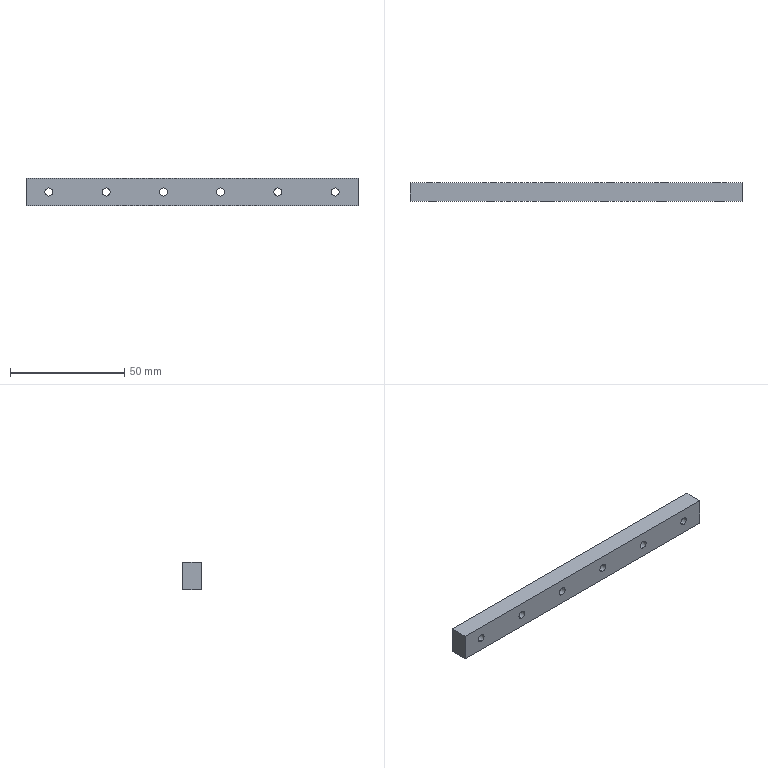Component | SolidWorks | MGN12H1R145Z0C-1_MGN12H145-1 | 1 solid | 36 faces | box 145 x 8 x 12 mm | volume 12955 mm3 | cylinder 24 | plane 12 | commonest cylinder face diameters 3.5 x12 6 x12 | material Plain Carbon Steel
build123d program:
from build123d import *

# Parameters (mm, degrees)
SKETCH1_W                                       = 12
SKETCH1_H                                       = 8
EXTRUDE1_DEPTH                                  = 145
M3_HEX_SOCKET_HEAD_CAP_SCREW_CBORE1_D           = 3.5
M3_HEX_SOCKET_HEAD_CAP_SCREW_CBORE1_CBORE_D     = 6
M3_HEX_SOCKET_HEAD_CAP_SCREW_CBORE1_CBORE_DEPTH = 4.5
LPATTERN1_COUNT                                 = 6
LPATTERN1_PITCH                                 = 25


with BuildPart() as part:
    # Sketch1 → Extrude1 (new body)
    with BuildSketch(Plane(origin=(0, 0, 0), x_dir=(0, 0, -1), z_dir=(1, 0, 0))):
        with Locations((0, 4)):
            Rectangle(SKETCH1_W, SKETCH1_H)
    extrude(amount=EXTRUDE1_DEPTH)

    # M3 Hex Socket Head Cap Screw CBORE1 (through all)
    with Locations(Plane(origin=(135, 8, 0), x_dir=(0, 0, 1), z_dir=(0, 1, 0))):
        with Locations((0, 0)):
            m3_hex_socket_head_cap_screw_cbore1 = CounterBoreHole(M3_HEX_SOCKET_HEAD_CAP_SCREW_CBORE1_D / 2, M3_HEX_SOCKET_HEAD_CAP_SCREW_CBORE1_CBORE_D / 2, M3_HEX_SOCKET_HEAD_CAP_SCREW_CBORE1_CBORE_DEPTH)

    # LPattern1: M3 Hex Socket Head Cap Screw CBORE1 ×6
    with Locations(*[(-i * LPATTERN1_PITCH, 0, 0) for i in range(1, LPATTERN1_COUNT)]):
        add(m3_hex_socket_head_cap_screw_cbore1, mode=Mode.SUBTRACT)


solid = part.part

# Placed as in the assembly
solid = solid.moved(Location((-3.73, 8.768, 38.329), (0, 0, 0)))
STEP:
#1=COLOUR_RGB('',0.7922,0.8196,0.9333);
#2=FILL_AREA_STYLE_COLOUR('',#1);
#3=FILL_AREA_STYLE('',(#2));
#4=SURFACE_STYLE_FILL_AREA(#3);
#5=SURFACE_SIDE_STYLE('',(#4));
#6=SURFACE_STYLE_USAGE(.BOTH.,#5);
#7=PRESENTATION_STYLE_ASSIGNMENT((#6));
#8=CARTESIAN_POINT('',(0.2469,0.3452,1.44));
#9=VERTEX_POINT('',#8);
#10=CARTESIAN_POINT('',(0.2469,0.3452,1.578));
#11=VERTEX_POINT('',#10);
#12=CARTESIAN_POINT('',(0.2469,0.3452,1.509));
#13=DIRECTION('',(0.,1.,0.));
#14=DIRECTION('',(0.,0.,1.));
#15=AXIS2_PLACEMENT_3D('',#12,#13,#14);
#16=CIRCLE('',#15,0.0689);
#17=EDGE_CURVE('',#9,#11,#16,.T.);
#18=ORIENTED_EDGE('',*,*,#17,.F.);
#19=CARTESIAN_POINT('',(0.2469,0.483,1.44));
#20=VERTEX_POINT('',#19);
#21=CARTESIAN_POINT('',(0.2469,0.6602,1.44));
#22=DIRECTION('',(0.,1.,0.));
#23=VECTOR('',#22,39.37);
#24=LINE('',#21,#23);
#25=EDGE_CURVE('',#9,#20,#24,.T.);
#26=ORIENTED_EDGE('',*,*,#25,.T.);
#27=CARTESIAN_POINT('',(0.2469,0.483,1.578));
#28=VERTEX_POINT('',#27);
#29=CARTESIAN_POINT('',(0.2469,0.483,1.509));
#30=DIRECTION('',(0.,1.,0.));
#31=DIRECTION('',(0.,0.,1.));
#32=AXIS2_PLACEMENT_3D('',#29,#30,#31);
#33=CIRCLE('',#32,0.0689);
#34=EDGE_CURVE('',#20,#28,#33,.T.);
#35=ORIENTED_EDGE('',*,*,#34,.T.);
#36=CARTESIAN_POINT('',(0.2469,0.6602,1.578));
#37=DIRECTION('',(0.,1.,0.));
#38=VECTOR('',#37,39.37);
#39=LINE('',#36,#38);
#40=EDGE_CURVE('',#11,#28,#39,.T.);
#41=ORIENTED_EDGE('',*,*,#40,.F.);
#42=EDGE_LOOP('',(#18,#26,#35,#41));
#43=FACE_OUTER_BOUND('',#42,.T.);
#44=CARTESIAN_POINT('',(0.2469,0.6602,1.509));
#45=DIRECTION('',(0.,1.,0.));
#46=DIRECTION('',(0.,0.,1.));
#47=AXIS2_PLACEMENT_3D('',#44,#45,#46);
#48=CYLINDRICAL_SURFACE('',#47,0.0689);
#49=ADVANCED_FACE('',(#43),#48,.F.);
#50=CARTESIAN_POINT('',(0.2469,0.483,1.391));
#51=VERTEX_POINT('',#50);
#52=CARTESIAN_POINT('',(0.2469,0.483,1.627));
#53=VERTEX_POINT('',#52);
#54=CARTESIAN_POINT('',(0.2469,0.483,1.509));
#55=DIRECTION('',(0.,1.,0.));
#56=DIRECTION('',(0.,0.,1.));
#57=AXIS2_PLACEMENT_3D('',#54,#55,#56);
#58=CIRCLE('',#57,0.1181);
#59=EDGE_CURVE('',#51,#53,#58,.T.);
#60=ORIENTED_EDGE('',*,*,#59,.F.);
#61=CARTESIAN_POINT('',(0.2469,0.6602,1.391));
#62=VERTEX_POINT('',#61);
#63=CARTESIAN_POINT('',(0.2469,0.6602,1.391));
#64=DIRECTION('',(0.,1.,0.));
#65=VECTOR('',#64,39.37);
#66=LINE('',#63,#65);
#67=EDGE_CURVE('',#51,#62,#66,.T.);
#68=ORIENTED_EDGE('',*,*,#67,.T.);
#69=CARTESIAN_POINT('',(0.2469,0.6602,1.627));
#70=VERTEX_POINT('',#69);
#71=CARTESIAN_POINT('',(0.2469,0.6602,1.509));
#72=DIRECTION('',(0.,1.,0.));
#73=DIRECTION('',(0.,0.,1.));
#74=AXIS2_PLACEMENT_3D('',#71,#72,#73);
#75=CIRCLE('',#74,0.1181);
#76=EDGE_CURVE('',#62,#70,#75,.T.);
#77=ORIENTED_EDGE('',*,*,#76,.T.);
#78=CARTESIAN_POINT('',(0.2469,0.6602,1.627));
#79=DIRECTION('',(0.,1.,0.));
#80=VECTOR('',#79,39.37);
#81=LINE('',#78,#80);
#82=EDGE_CURVE('',#53,#70,#81,.T.);
#83=ORIENTED_EDGE('',*,*,#82,.F.);
#84=EDGE_LOOP('',(#60,#68,#77,#83));
#85=FACE_OUTER_BOUND('',#84,.T.);
#86=CARTESIAN_POINT('',(0.2469,0.6602,1.509));
#87=DIRECTION('',(0.,1.,0.));
#88=DIRECTION('',(0.,0.,1.));
#89=AXIS2_PLACEMENT_3D('',#86,#87,#88);
#90=CYLINDRICAL_SURFACE('',#89,0.1181);
#91=ADVANCED_FACE('',(#85),#90,.F.);
#92=CARTESIAN_POINT('',(1.231,0.3452,1.44));
#93=VERTEX_POINT('',#92);
#94=CARTESIAN_POINT('',(1.231,0.3452,1.578));
#95=VERTEX_POINT('',#94);
#96=CARTESIAN_POINT('',(1.231,0.3452,1.509));
#97=DIRECTION('',(0.,1.,0.));
#98=DIRECTION('',(0.,0.,1.));
#99=AXIS2_PLACEMENT_3D('',#96,#97,#98);
#100=CIRCLE('',#99,0.0689);
#101=EDGE_CURVE('',#93,#95,#100,.T.);
#102=ORIENTED_EDGE('',*,*,#101,.F.);
#103=CARTESIAN_POINT('',(1.231,0.483,1.44));
#104=VERTEX_POINT('',#103);
#105=CARTESIAN_POINT('',(1.231,0.6602,1.44));
#106=DIRECTION('',(0.,1.,0.));
#107=VECTOR('',#106,39.37);
#108=LINE('',#105,#107);
#109=EDGE_CURVE('',#93,#104,#108,.T.);
#110=ORIENTED_EDGE('',*,*,#109,.T.);
#111=CARTESIAN_POINT('',(1.231,0.483,1.578));
#112=VERTEX_POINT('',#111);
#113=CARTESIAN_POINT('',(1.231,0.483,1.509));
#114=DIRECTION('',(0.,1.,0.));
#115=DIRECTION('',(0.,0.,1.));
#116=AXIS2_PLACEMENT_3D('',#113,#114,#115);
#117=CIRCLE('',#116,0.0689);
#118=EDGE_CURVE('',#104,#112,#117,.T.);
#119=ORIENTED_EDGE('',*,*,#118,.T.);
#120=CARTESIAN_POINT('',(1.231,0.6602,1.578));
#121=DIRECTION('',(0.,1.,0.));
#122=VECTOR('',#121,39.37);
#123=LINE('',#120,#122);
#124=EDGE_CURVE('',#95,#112,#123,.T.);
#125=ORIENTED_EDGE('',*,*,#124,.F.);
#126=EDGE_LOOP('',(#102,#110,#119,#125));
#127=FACE_OUTER_BOUND('',#126,.T.);
#128=CARTESIAN_POINT('',(1.231,0.6602,1.509));
#129=DIRECTION('',(0.,1.,0.));
#130=DIRECTION('',(0.,0.,1.));
#131=AXIS2_PLACEMENT_3D('',#128,#129,#130);
#132=CYLINDRICAL_SURFACE('',#131,0.0689);
#133=ADVANCED_FACE('',(#127),#132,.F.);
#134=CARTESIAN_POINT('',(1.231,0.483,1.391));
#135=VERTEX_POINT('',#134);
#136=CARTESIAN_POINT('',(1.231,0.483,1.627));
#137=VERTEX_POINT('',#136);
#138=CARTESIAN_POINT('',(1.231,0.483,1.509));
#139=DIRECTION('',(0.,1.,0.));
#140=DIRECTION('',(0.,0.,1.));
#141=AXIS2_PLACEMENT_3D('',#138,#139,#140);
#142=CIRCLE('',#141,0.1181);
#143=EDGE_CURVE('',#135,#137,#142,.T.);
#144=ORIENTED_EDGE('',*,*,#143,.F.);
#145=CARTESIAN_POINT('',(1.231,0.6602,1.391));
#146=VERTEX_POINT('',#145);
#147=CARTESIAN_POINT('',(1.231,0.6602,1.391));
#148=DIRECTION('',(0.,1.,0.));
#149=VECTOR('',#148,39.37);
#150=LINE('',#147,#149);
#151=EDGE_CURVE('',#135,#146,#150,.T.);
#152=ORIENTED_EDGE('',*,*,#151,.T.);
#153=CARTESIAN_POINT('',(1.231,0.6602,1.627));
#154=VERTEX_POINT('',#153);
#155=CARTESIAN_POINT('',(1.231,0.6602,1.509));
#156=DIRECTION('',(0.,1.,0.));
#157=DIRECTION('',(0.,0.,1.));
#158=AXIS2_PLACEMENT_3D('',#155,#156,#157);
#159=CIRCLE('',#158,0.1181);
#160=EDGE_CURVE('',#146,#154,#159,.T.);
#161=ORIENTED_EDGE('',*,*,#160,.T.);
#162=CARTESIAN_POINT('',(1.231,0.6602,1.627));
#163=DIRECTION('',(0.,1.,0.));
#164=VECTOR('',#163,39.37);
#165=LINE('',#162,#164);
#166=EDGE_CURVE('',#137,#154,#165,.T.);
#167=ORIENTED_EDGE('',*,*,#166,.F.);
#168=EDGE_LOOP('',(#144,#152,#161,#167));
#169=FACE_OUTER_BOUND('',#168,.T.);
#170=CARTESIAN_POINT('',(1.231,0.6602,1.509));
#171=DIRECTION('',(0.,1.,0.));
#172=DIRECTION('',(0.,0.,1.));
#173=AXIS2_PLACEMENT_3D('',#170,#171,#172);
#174=CYLINDRICAL_SURFACE('',#173,0.1181);
#175=ADVANCED_FACE('',(#169),#174,.F.);
#176=CARTESIAN_POINT('',(2.215,0.3452,1.44));
#177=VERTEX_POINT('',#176);
#178=CARTESIAN_POINT('',(2.215,0.3452,1.578));
#179=VERTEX_POINT('',#178);
#180=CARTESIAN_POINT('',(2.215,0.3452,1.509));
#181=DIRECTION('',(0.,1.,0.));
#182=DIRECTION('',(0.,0.,1.));
#183=AXIS2_PLACEMENT_3D('',#180,#181,#182);
#184=CIRCLE('',#183,0.0689);
#185=EDGE_CURVE('',#177,#179,#184,.T.);
#186=ORIENTED_EDGE('',*,*,#185,.F.);
#187=CARTESIAN_POINT('',(2.215,0.483,1.44));
#188=VERTEX_POINT('',#187);
#189=CARTESIAN_POINT('',(2.215,0.6602,1.44));
#190=DIRECTION('',(0.,1.,0.));
#191=VECTOR('',#190,39.37);
#192=LINE('',#189,#191);
#193=EDGE_CURVE('',#177,#188,#192,.T.);
#194=ORIENTED_EDGE('',*,*,#193,.T.);
#195=CARTESIAN_POINT('',(2.215,0.483,1.578));
#196=VERTEX_POINT('',#195);
#197=CARTESIAN_POINT('',(2.215,0.483,1.509));
#198=DIRECTION('',(0.,1.,0.));
#199=DIRECTION('',(0.,0.,1.));
#200=AXIS2_PLACEMENT_3D('',#197,#198,#199);
#201=CIRCLE('',#200,0.0689);
#202=EDGE_CURVE('',#188,#196,#201,.T.);
#203=ORIENTED_EDGE('',*,*,#202,.T.);
#204=CARTESIAN_POINT('',(2.215,0.6602,1.578));
#205=DIRECTION('',(0.,1.,0.));
#206=VECTOR('',#205,39.37);
#207=LINE('',#204,#206);
#208=EDGE_CURVE('',#179,#196,#207,.T.);
#209=ORIENTED_EDGE('',*,*,#208,.F.);
#210=EDGE_LOOP('',(#186,#194,#203,#209));
#211=FACE_OUTER_BOUND('',#210,.T.);
#212=CARTESIAN_POINT('',(2.215,0.6602,1.509));
#213=DIRECTION('',(0.,1.,0.));
#214=DIRECTION('',(0.,0.,1.));
#215=AXIS2_PLACEMENT_3D('',#212,#213,#214);
#216=CYLINDRICAL_SURFACE('',#215,0.0689);
#217=ADVANCED_FACE('',(#211),#216,.F.);
#218=CARTESIAN_POINT('',(2.215,0.483,1.391));
#219=VERTEX_POINT('',#218);
#220=CARTESIAN_POINT('',(2.215,0.483,1.627));
#221=VERTEX_POINT('',#220);
#222=CARTESIAN_POINT('',(2.215,0.483,1.509));
#223=DIRECTION('',(0.,1.,0.));
#224=DIRECTION('',(0.,0.,1.));
#225=AXIS2_PLACEMENT_3D('',#222,#223,#224);
#226=CIRCLE('',#225,0.1181);
#227=EDGE_CURVE('',#219,#221,#226,.T.);
#228=ORIENTED_EDGE('',*,*,#227,.F.);
#229=CARTESIAN_POINT('',(2.215,0.6602,1.391));
#230=VERTEX_POINT('',#229);
#231=CARTESIAN_POINT('',(2.215,0.6602,1.391));
#232=DIRECTION('',(0.,1.,0.));
#233=VECTOR('',#232,39.37);
#234=LINE('',#231,#233);
#235=EDGE_CURVE('',#219,#230,#234,.T.);
#236=ORIENTED_EDGE('',*,*,#235,.T.);
#237=CARTESIAN_POINT('',(2.215,0.6602,1.627));
#238=VERTEX_POINT('',#237);
#239=CARTESIAN_POINT('',(2.215,0.6602,1.509));
#240=DIRECTION('',(0.,1.,0.));
#241=DIRECTION('',(0.,0.,1.));
#242=AXIS2_PLACEMENT_3D('',#239,#240,#241);
#243=CIRCLE('',#242,0.1181);
#244=EDGE_CURVE('',#230,#238,#243,.T.);
#245=ORIENTED_EDGE('',*,*,#244,.T.);
#246=CARTESIAN_POINT('',(2.215,0.6602,1.627));
#247=DIRECTION('',(0.,1.,0.));
#248=VECTOR('',#247,39.37);
#249=LINE('',#246,#248);
#250=EDGE_CURVE('',#221,#238,#249,.T.);
#251=ORIENTED_EDGE('',*,*,#250,.F.);
#252=EDGE_LOOP('',(#228,#236,#245,#251));
#253=FACE_OUTER_BOUND('',#252,.T.);
#254=CARTESIAN_POINT('',(2.215,0.6602,1.509));
#255=DIRECTION('',(0.,1.,0.));
#256=DIRECTION('',(0.,0.,1.));
#257=AXIS2_PLACEMENT_3D('',#254,#255,#256);
#258=CYLINDRICAL_SURFACE('',#257,0.1181);
#259=ADVANCED_FACE('',(#253),#258,.F.);
#260=CARTESIAN_POINT('',(3.2,0.3452,1.44));
#261=VERTEX_POINT('',#260);
#262=CARTESIAN_POINT('',(3.2,0.3452,1.578));
#263=VERTEX_POINT('',#262);
#264=CARTESIAN_POINT('',(3.2,0.3452,1.509));
#265=DIRECTION('',(0.,1.,0.));
#266=DIRECTION('',(0.,0.,1.));
#267=AXIS2_PLACEMENT_3D('',#264,#265,#266);
#268=CIRCLE('',#267,0.0689);
#269=EDGE_CURVE('',#261,#263,#268,.T.);
#270=ORIENTED_EDGE('',*,*,#269,.F.);
#271=CARTESIAN_POINT('',(3.2,0.483,1.44));
#272=VERTEX_POINT('',#271);
#273=CARTESIAN_POINT('',(3.2,0.6602,1.44));
#274=DIRECTION('',(0.,1.,0.));
#275=VECTOR('',#274,39.37);
#276=LINE('',#273,#275);
#277=EDGE_CURVE('',#261,#272,#276,.T.);
#278=ORIENTED_EDGE('',*,*,#277,.T.);
#279=CARTESIAN_POINT('',(3.2,0.483,1.578));
#280=VERTEX_POINT('',#279);
#281=CARTESIAN_POINT('',(3.2,0.483,1.509));
#282=DIRECTION('',(0.,1.,0.));
#283=DIRECTION('',(0.,0.,1.));
#284=AXIS2_PLACEMENT_3D('',#281,#282,#283);
#285=CIRCLE('',#284,0.0689);
#286=EDGE_CURVE('',#272,#280,#285,.T.);
#287=ORIENTED_EDGE('',*,*,#286,.T.);
#288=CARTESIAN_POINT('',(3.2,0.6602,1.578));
#289=DIRECTION('',(0.,1.,0.));
#290=VECTOR('',#289,39.37);
#291=LINE('',#288,#290);
#292=EDGE_CURVE('',#263,#280,#291,.T.);
#293=ORIENTED_EDGE('',*,*,#292,.F.);
#294=EDGE_LOOP('',(#270,#278,#287,#293));
#295=FACE_OUTER_BOUND('',#294,.T.);
#296=CARTESIAN_POINT('',(3.2,0.6602,1.509));
#297=DIRECTION('',(0.,1.,0.));
#298=DIRECTION('',(0.,0.,1.));
#299=AXIS2_PLACEMENT_3D('',#296,#297,#298);
#300=CYLINDRICAL_SURFACE('',#299,0.0689);
#301=ADVANCED_FACE('',(#295),#300,.F.);
#302=CARTESIAN_POINT('',(3.2,0.483,1.391));
#303=VERTEX_POINT('',#302);
#304=CARTESIAN_POINT('',(3.2,0.483,1.627));
#305=VERTEX_POINT('',#304);
#306=CARTESIAN_POINT('',(3.2,0.483,1.509));
#307=DIRECTION('',(0.,1.,0.));
#308=DIRECTION('',(0.,0.,1.));
#309=AXIS2_PLACEMENT_3D('',#306,#307,#308);
#310=CIRCLE('',#309,0.1181);
#311=EDGE_CURVE('',#303,#305,#310,.T.);
#312=ORIENTED_EDGE('',*,*,#311,.F.);
#313=CARTESIAN_POINT('',(3.2,0.6602,1.391));
#314=VERTEX_POINT('',#313);
#315=CARTESIAN_POINT('',(3.2,0.6602,1.391));
#316=DIRECTION('',(0.,1.,0.));
#317=VECTOR('',#316,39.37);
#318=LINE('',#315,#317);
#319=EDGE_CURVE('',#303,#314,#318,.T.);
#320=ORIENTED_EDGE('',*,*,#319,.T.);
#321=CARTESIAN_POINT('',(3.2,0.6602,1.627));
#322=VERTEX_POINT('',#321);
#323=CARTESIAN_POINT('',(3.2,0.6602,1.509));
#324=DIRECTION('',(0.,1.,0.));
#325=DIRECTION('',(0.,0.,1.));
#326=AXIS2_PLACEMENT_3D('',#323,#324,#325);
#327=CIRCLE('',#326,0.1181);
#328=EDGE_CURVE('',#314,#322,#327,.T.);
#329=ORIENTED_EDGE('',*,*,#328,.T.);
#330=CARTESIAN_POINT('',(3.2,0.6602,1.627));
#331=DIRECTION('',(0.,1.,0.));
#332=VECTOR('',#331,39.37);
#333=LINE('',#330,#332);
#334=EDGE_CURVE('',#305,#322,#333,.T.);
#335=ORIENTED_EDGE('',*,*,#334,.F.);
#336=EDGE_LOOP('',(#312,#320,#329,#335));
#337=FACE_OUTER_BOUND('',#336,.T.);
#338=CARTESIAN_POINT('',(3.2,0.6602,1.509));
#339=DIRECTION('',(0.,1.,0.));
#340=DIRECTION('',(0.,0.,1.));
#341=AXIS2_PLACEMENT_3D('',#338,#339,#340);
#342=CYLINDRICAL_SURFACE('',#341,0.1181);
#343=ADVANCED_FACE('',(#337),#342,.F.);
#344=CARTESIAN_POINT('',(4.184,0.3452,1.44));
#345=VERTEX_POINT('',#344);
#346=CARTESIAN_POINT('',(4.184,0.3452,1.578));
#347=VERTEX_POINT('',#346);
#348=CARTESIAN_POINT('',(4.184,0.3452,1.509));
#349=DIRECTION('',(0.,1.,0.));
#350=DIRECTION('',(0.,0.,1.));
#351=AXIS2_PLACEMENT_3D('',#348,#349,#350);
#352=CIRCLE('',#351,0.0689);
#353=EDGE_CURVE('',#345,#347,#352,.T.);
#354=ORIENTED_EDGE('',*,*,#353,.F.);
#355=CARTESIAN_POINT('',(4.184,0.483,1.44));
#356=VERTEX_POINT('',#355);
#357=CARTESIAN_POINT('',(4.184,0.6602,1.44));
#358=DIRECTION('',(0.,1.,0.));
#359=VECTOR('',#358,39.37);
#360=LINE('',#357,#359);
#361=EDGE_CURVE('',#345,#356,#360,.T.);
#362=ORIENTED_EDGE('',*,*,#361,.T.);
#363=CARTESIAN_POINT('',(4.184,0.483,1.578));
#364=VERTEX_POINT('',#363);
#365=CARTESIAN_POINT('',(4.184,0.483,1.509));
#366=DIRECTION('',(0.,1.,0.));
#367=DIRECTION('',(0.,0.,1.));
#368=AXIS2_PLACEMENT_3D('',#365,#366,#367);
#369=CIRCLE('',#368,0.0689);
#370=EDGE_CURVE('',#356,#364,#369,.T.);
#371=ORIENTED_EDGE('',*,*,#370,.T.);
#372=CARTESIAN_POINT('',(4.184,0.6602,1.578));
#373=DIRECTION('',(0.,1.,0.));
#374=VECTOR('',#373,39.37);
#375=LINE('',#372,#374);
#376=EDGE_CURVE('',#347,#364,#375,.T.);
#377=ORIENTED_EDGE('',*,*,#376,.F.);
#378=EDGE_LOOP('',(#354,#362,#371,#377));
#379=FACE_OUTER_BOUND('',#378,.T.);
#380=CARTESIAN_POINT('',(4.184,0.6602,1.509));
#381=DIRECTION('',(0.,1.,0.));
#382=DIRECTION('',(0.,0.,1.));
#383=AXIS2_PLACEMENT_3D('',#380,#381,#382);
#384=CYLINDRICAL_SURFACE('',#383,0.0689);
#385=ADVANCED_FACE('',(#379),#384,.F.);
#386=CARTESIAN_POINT('',(4.184,0.483,1.391));
#387=VERTEX_POINT('',#386);
#388=CARTESIAN_POINT('',(4.184,0.483,1.627));
#389=VERTEX_POINT('',#388);
#390=CARTESIAN_POINT('',(4.184,0.483,1.509));
#391=DIRECTION('',(0.,1.,0.));
#392=DIRECTION('',(0.,0.,1.));
#393=AXIS2_PLACEMENT_3D('',#390,#391,#392);
#394=CIRCLE('',#393,0.1181);
#395=EDGE_CURVE('',#387,#389,#394,.T.);
#396=ORIENTED_EDGE('',*,*,#395,.F.);
#397=CARTESIAN_POINT('',(4.184,0.6602,1.391));
#398=VERTEX_POINT('',#397);
#399=CARTESIAN_POINT('',(4.184,0.6602,1.391));
#400=DIRECTION('',(0.,1.,0.));
#401=VECTOR('',#400,39.37);
#402=LINE('',#399,#401);
#403=EDGE_CURVE('',#387,#398,#402,.T.);
#404=ORIENTED_EDGE('',*,*,#403,.T.);
#405=CARTESIAN_POINT('',(4.184,0.6602,1.627));
#406=VERTEX_POINT('',#405);
#407=CARTESIAN_POINT('',(4.184,0.6602,1.509));
#408=DIRECTION('',(0.,1.,0.));
#409=DIRECTION('',(0.,0.,1.));
#410=AXIS2_PLACEMENT_3D('',#407,#408,#409);
#411=CIRCLE('',#410,0.1181);
#412=EDGE_CURVE('',#398,#406,#411,.T.);
#413=ORIENTED_EDGE('',*,*,#412,.T.);
#414=CARTESIAN_POINT('',(4.184,0.6602,1.627));
#415=DIRECTION('',(0.,1.,0.));
#416=VECTOR('',#415,39.37);
#417=LINE('',#414,#416);
#418=EDGE_CURVE('',#389,#406,#417,.T.);
#419=ORIENTED_EDGE('',*,*,#418,.F.);
#420=EDGE_LOOP('',(#396,#404,#413,#419));
#421=FACE_OUTER_BOUND('',#420,.T.);
#422=CARTESIAN_POINT('',(4.184,0.6602,1.509));
#423=DIRECTION('',(0.,1.,0.));
#424=DIRECTION('',(0.,0.,1.));
#425=AXIS2_PLACEMENT_3D('',#422,#423,#424);
#426=CYLINDRICAL_SURFACE('',#425,0.1181);
#427=ADVANCED_FACE('',(#421),#426,.F.);
#428=CARTESIAN_POINT('',(5.168,0.3452,1.44));
#429=VERTEX_POINT('',#428);
#430=CARTESIAN_POINT('',(5.168,0.3452,1.578));
#431=VERTEX_POINT('',#430);
#432=CARTESIAN_POINT('',(5.168,0.3452,1.509));
#433=DIRECTION('',(0.,1.,0.));
#434=DIRECTION('',(0.,0.,1.));
#435=AXIS2_PLACEMENT_3D('',#432,#433,#434);
#436=CIRCLE('',#435,0.0689);
#437=EDGE_CURVE('',#429,#431,#436,.T.);
#438=ORIENTED_EDGE('',*,*,#437,.F.);
#439=CARTESIAN_POINT('',(5.168,0.483,1.44));
#440=VERTEX_POINT('',#439);
#441=CARTESIAN_POINT('',(5.168,0.6602,1.44));
#442=DIRECTION('',(0.,1.,0.));
#443=VECTOR('',#442,39.37);
#444=LINE('',#441,#443);
#445=EDGE_CURVE('',#429,#440,#444,.T.);
#446=ORIENTED_EDGE('',*,*,#445,.T.);
#447=CARTESIAN_POINT('',(5.168,0.483,1.578));
#448=VERTEX_POINT('',#447);
#449=CARTESIAN_POINT('',(5.168,0.483,1.509));
#450=DIRECTION('',(0.,1.,0.));
#451=DIRECTION('',(0.,0.,1.));
#452=AXIS2_PLACEMENT_3D('',#449,#450,#451);
#453=CIRCLE('',#452,0.0689);
#454=EDGE_CURVE('',#440,#448,#453,.T.);
#455=ORIENTED_EDGE('',*,*,#454,.T.);
#456=CARTESIAN_POINT('',(5.168,0.6602,1.578));
#457=DIRECTION('',(0.,1.,0.));
#458=VECTOR('',#457,39.37);
#459=LINE('',#456,#458);
#460=EDGE_CURVE('',#431,#448,#459,.T.);
#461=ORIENTED_EDGE('',*,*,#460,.F.);
#462=EDGE_LOOP('',(#438,#446,#455,#461));
#463=FACE_OUTER_BOUND('',#462,.T.);
#464=CARTESIAN_POINT('',(5.168,0.6602,1.509));
#465=DIRECTION('',(0.,1.,0.));
#466=DIRECTION('',(0.,0.,1.));
#467=AXIS2_PLACEMENT_3D('',#464,#465,#466);
#468=CYLINDRICAL_SURFACE('',#467,0.0689);
#469=ADVANCED_FACE('',(#463),#468,.F.);
#470=CARTESIAN_POINT('',(5.168,0.483,1.391));
#471=VERTEX_POINT('',#470);
#472=CARTESIAN_POINT('',(5.168,0.483,1.627));
#473=VERTEX_POINT('',#472);
#474=CARTESIAN_POINT('',(5.168,0.483,1.509));
#475=DIRECTION('',(0.,1.,0.));
#476=DIRECTION('',(0.,0.,1.));
#477=AXIS2_PLACEMENT_3D('',#474,#475,#476);
#478=CIRCLE('',#477,0.1181);
#479=EDGE_CURVE('',#471,#473,#478,.T.);
#480=ORIENTED_EDGE('',*,*,#479,.F.);
#481=CARTESIAN_POINT('',(5.168,0.6602,1.391));
#482=VERTEX_POINT('',#481);
#483=CARTESIAN_POINT('',(5.168,0.6602,1.391));
#484=DIRECTION('',(0.,1.,0.));
#485=VECTOR('',#484,39.37);
#486=LINE('',#483,#485);
#487=EDGE_CURVE('',#471,#482,#486,.T.);
#488=ORIENTED_EDGE('',*,*,#487,.T.);
#489=CARTESIAN_POINT('',(5.168,0.6602,1.627));
#490=VERTEX_POINT('',#489);
#491=CARTESIAN_POINT('',(5.168,0.6602,1.509));
#492=DIRECTION('',(0.,1.,0.));
#493=DIRECTION('',(0.,0.,1.));
#494=AXIS2_PLACEMENT_3D('',#491,#492,#493);
#495=CIRCLE('',#494,0.1181);
#496=EDGE_CURVE('',#482,#490,#495,.T.);
#497=ORIENTED_EDGE('',*,*,#496,.T.);
#498=CARTESIAN_POINT('',(5.168,0.6602,1.627));
#499=DIRECTION('',(0.,1.,0.));
#500=VECTOR('',#499,39.37);
#501=LINE('',#498,#500);
#502=EDGE_CURVE('',#473,#490,#501,.T.);
#503=ORIENTED_EDGE('',*,*,#502,.F.);
#504=EDGE_LOOP('',(#480,#488,#497,#503));
#505=FACE_OUTER_BOUND('',#504,.T.);
#506=CARTESIAN_POINT('',(5.168,0.6602,1.509));
#507=DIRECTION('',(0.,1.,0.));
#508=DIRECTION('',(0.,0.,1.));
#509=AXIS2_PLACEMENT_3D('',#506,#507,#508);
#510=CYLINDRICAL_SURFACE('',#509,0.1181);
#511=ADVANCED_FACE('',(#505),#510,.F.);
#512=CARTESIAN_POINT('',(0.2469,0.6602,1.509));
#513=DIRECTION('',(0.,1.,0.));
#514=DIRECTION('',(0.,0.,1.));
#515=AXIS2_PLACEMENT_3D('',#512,#513,#514);
#516=CIRCLE('',#515,0.1181);
#517=EDGE_CURVE('',#70,#62,#516,.T.);
#518=ORIENTED_EDGE('',*,*,#517,.F.);
#519=ORIENTED_EDGE('',*,*,#76,.F.);
#520=EDGE_LOOP('',(#518,#519));
#521=FACE_BOUND('',#520,.T.);
#522=CARTESIAN_POINT('',(1.231,0.6602,1.509));
#523=DIRECTION('',(0.,1.,0.));
#524=DIRECTION('',(0.,0.,1.));
#525=AXIS2_PLACEMENT_3D('',#522,#523,#524);
#526=CIRCLE('',#525,0.1181);
#527=EDGE_CURVE('',#154,#146,#526,.T.);
#528=ORIENTED_EDGE('',*,*,#527,.F.);
#529=ORIENTED_EDGE('',*,*,#160,.F.);
#530=EDGE_LOOP('',(#528,#529));
#531=FACE_BOUND('',#530,.T.);
#532=CARTESIAN_POINT('',(2.215,0.6602,1.509));
#533=DIRECTION('',(0.,1.,0.));
#534=DIRECTION('',(0.,0.,1.));
#535=AXIS2_PLACEMENT_3D('',#532,#533,#534);
#536=CIRCLE('',#535,0.1181);
#537=EDGE_CURVE('',#238,#230,#536,.T.);
#538=ORIENTED_EDGE('',*,*,#537,.F.);
#539=ORIENTED_EDGE('',*,*,#244,.F.);
#540=EDGE_LOOP('',(#538,#539));
#541=FACE_BOUND('',#540,.T.);
#542=CARTESIAN_POINT('',(4.184,0.6602,1.509));
#543=DIRECTION('',(0.,1.,0.));
#544=DIRECTION('',(0.,0.,1.));
#545=AXIS2_PLACEMENT_3D('',#542,#543,#544);
#546=CIRCLE('',#545,0.1181);
#547=EDGE_CURVE('',#406,#398,#546,.T.);
#548=ORIENTED_EDGE('',*,*,#547,.F.);
#549=ORIENTED_EDGE('',*,*,#412,.F.);
#550=EDGE_LOOP('',(#548,#549));
#551=FACE_BOUND('',#550,.T.);
#552=CARTESIAN_POINT('',(5.168,0.6602,1.509));
#553=DIRECTION('',(0.,1.,0.));
#554=DIRECTION('',(0.,0.,1.));
#555=AXIS2_PLACEMENT_3D('',#552,#553,#554);
#556=CIRCLE('',#555,0.1181);
#557=EDGE_CURVE('',#490,#482,#556,.T.);
#558=ORIENTED_EDGE('',*,*,#557,.F.);
#559=ORIENTED_EDGE('',*,*,#496,.F.);
#560=EDGE_LOOP('',(#558,#559));
#561=FACE_BOUND('',#560,.T.);
#562=CARTESIAN_POINT('',(-0.1468,0.6602,1.273));
#563=VERTEX_POINT('',#562);
#564=CARTESIAN_POINT('',(-0.1468,0.6602,1.745));
#565=VERTEX_POINT('',#564);
#566=CARTESIAN_POINT('',(-0.1468,0.6602,1.745));
#567=DIRECTION('',(0.,0.,1.));
#568=VECTOR('',#567,39.37);
#569=LINE('',#566,#568);
#570=EDGE_CURVE('',#563,#565,#569,.T.);
#571=ORIENTED_EDGE('',*,*,#570,.T.);
#572=CARTESIAN_POINT('',(5.562,0.6602,1.745));
#573=VERTEX_POINT('',#572);
#574=CARTESIAN_POINT('',(5.562,0.6602,1.745));
#575=DIRECTION('',(-1.,0.,0.));
#576=VECTOR('',#575,39.37);
#577=LINE('',#574,#576);
#578=EDGE_CURVE('',#573,#565,#577,.T.);
#579=ORIENTED_EDGE('',*,*,#578,.F.);
#580=CARTESIAN_POINT('',(5.562,0.6602,1.273));
#581=VERTEX_POINT('',#580);
#582=CARTESIAN_POINT('',(5.562,0.6602,1.745));
#583=DIRECTION('',(0.,0.,1.));
#584=VECTOR('',#583,39.37);
#585=LINE('',#582,#584);
#586=EDGE_CURVE('',#581,#573,#585,.T.);
#587=ORIENTED_EDGE('',*,*,#586,.F.);
#588=CARTESIAN_POINT('',(5.562,0.6602,1.273));
#589=DIRECTION('',(-1.,0.,0.));
#590=VECTOR('',#589,39.37);
#591=LINE('',#588,#590);
#592=EDGE_CURVE('',#581,#563,#591,.T.);
#593=ORIENTED_EDGE('',*,*,#592,.T.);
#594=EDGE_LOOP('',(#571,#579,#587,#593));
#595=FACE_OUTER_BOUND('',#594,.T.);
#596=CARTESIAN_POINT('',(3.2,0.6602,1.509));
#597=DIRECTION('',(0.,1.,0.));
#598=DIRECTION('',(0.,0.,1.));
#599=AXIS2_PLACEMENT_3D('',#596,#597,#598);
#600=CIRCLE('',#599,0.1181);
#601=EDGE_CURVE('',#322,#314,#600,.T.);
#602=ORIENTED_EDGE('',*,*,#601,.F.);
#603=ORIENTED_EDGE('',*,*,#328,.F.);
#604=EDGE_LOOP('',(#602,#603));
#605=FACE_BOUND('',#604,.T.);
#606=CARTESIAN_POINT('',(5.562,0.6602,1.745));
#607=DIRECTION('',(0.,-1.,0.));
#608=DIRECTION('',(0.,0.,-1.));
#609=AXIS2_PLACEMENT_3D('',#606,#607,#608);
#610=PLANE('',#609);
#611=ADVANCED_FACE('',(#521,#531,#541,#551,#561,#595,#605),#610,.F.);
#612=CARTESIAN_POINT('',(-0.1468,0.3452,1.745));
#613=VERTEX_POINT('',#612);
#614=CARTESIAN_POINT('',(-0.1468,0.6602,1.745));
#615=DIRECTION('',(0.,-1.,-0.));
#616=VECTOR('',#615,39.37);
#617=LINE('',#614,#616);
#618=EDGE_CURVE('',#565,#613,#617,.T.);
#619=ORIENTED_EDGE('',*,*,#618,.T.);
#620=CARTESIAN_POINT('',(5.562,0.3452,1.745));
#621=VERTEX_POINT('',#620);
#622=CARTESIAN_POINT('',(5.562,0.3452,1.745));
#623=DIRECTION('',(-1.,0.,0.));
#624=VECTOR('',#623,39.37);
#625=LINE('',#622,#624);
#626=EDGE_CURVE('',#621,#613,#625,.T.);
#627=ORIENTED_EDGE('',*,*,#626,.F.);
#628=CARTESIAN_POINT('',(5.562,0.6602,1.745));
#629=DIRECTION('',(0.,-1.,-0.));
#630=VECTOR('',#629,39.37);
#631=LINE('',#628,#630);
#632=EDGE_CURVE('',#573,#621,#631,.T.);
#633=ORIENTED_EDGE('',*,*,#632,.F.);
#634=ORIENTED_EDGE('',*,*,#578,.T.);
#635=EDGE_LOOP('',(#619,#627,#633,#634));
#636=FACE_OUTER_BOUND('',#635,.T.);
#637=CARTESIAN_POINT('',(5.562,0.6602,1.745));
#638=DIRECTION('',(0.,0.,-1.));
#639=DIRECTION('',(0.,1.,0.));
#640=AXIS2_PLACEMENT_3D('',#637,#638,#639);
#641=PLANE('',#640);
#642=ADVANCED_FACE('',(#636),#641,.F.);
#643=CARTESIAN_POINT('',(0.2469,0.3452,1.509));
#644=DIRECTION('',(0.,1.,0.));
#645=DIRECTION('',(0.,0.,1.));
#646=AXIS2_PLACEMENT_3D('',#643,#644,#645);
#647=CIRCLE('',#646,0.0689);
#648=EDGE_CURVE('',#11,#9,#647,.T.);
#649=ORIENTED_EDGE('',*,*,#648,.T.);
#650=ORIENTED_EDGE('',*,*,#17,.T.);
#651=EDGE_LOOP('',(#649,#650));
#652=FACE_BOUND('',#651,.T.);
#653=CARTESIAN_POINT('',(1.231,0.3452,1.509));
#654=DIRECTION('',(0.,1.,0.));
#655=DIRECTION('',(0.,0.,1.));
#656=AXIS2_PLACEMENT_3D('',#653,#654,#655);
#657=CIRCLE('',#656,0.0689);
#658=EDGE_CURVE('',#95,#93,#657,.T.);
#659=ORIENTED_EDGE('',*,*,#658,.T.);
#660=ORIENTED_EDGE('',*,*,#101,.T.);
#661=EDGE_LOOP('',(#659,#660));
#662=FACE_BOUND('',#661,.T.);
#663=CARTESIAN_POINT('',(2.215,0.3452,1.509));
#664=DIRECTION('',(0.,1.,0.));
#665=DIRECTION('',(0.,0.,1.));
#666=AXIS2_PLACEMENT_3D('',#663,#664,#665);
#667=CIRCLE('',#666,0.0689);
#668=EDGE_CURVE('',#179,#177,#667,.T.);
#669=ORIENTED_EDGE('',*,*,#668,.T.);
#670=ORIENTED_EDGE('',*,*,#185,.T.);
#671=EDGE_LOOP('',(#669,#670));
#672=FACE_BOUND('',#671,.T.);
#673=CARTESIAN_POINT('',(3.2,0.3452,1.509));
#674=DIRECTION('',(0.,1.,0.));
#675=DIRECTION('',(0.,0.,1.));
#676=AXIS2_PLACEMENT_3D('',#673,#674,#675);
#677=CIRCLE('',#676,0.0689);
#678=EDGE_CURVE('',#263,#261,#677,.T.);
#679=ORIENTED_EDGE('',*,*,#678,.T.);
#680=ORIENTED_EDGE('',*,*,#269,.T.);
#681=EDGE_LOOP('',(#679,#680));
#682=FACE_BOUND('',#681,.T.);
#683=CARTESIAN_POINT('',(4.184,0.3452,1.509));
#684=DIRECTION('',(0.,1.,0.));
#685=DIRECTION('',(0.,0.,1.));
#686=AXIS2_PLACEMENT_3D('',#683,#684,#685);
#687=CIRCLE('',#686,0.0689);
#688=EDGE_CURVE('',#347,#345,#687,.T.);
#689=ORIENTED_EDGE('',*,*,#688,.T.);
#690=ORIENTED_EDGE('',*,*,#353,.T.);
#691=EDGE_LOOP('',(#689,#690));
#692=FACE_BOUND('',#691,.T.);
#693=CARTESIAN_POINT('',(5.168,0.3452,1.509));
#694=DIRECTION('',(0.,1.,0.));
#695=DIRECTION('',(0.,0.,1.));
#696=AXIS2_PLACEMENT_3D('',#693,#694,#695);
#697=CIRCLE('',#696,0.0689);
#698=EDGE_CURVE('',#431,#429,#697,.T.);
#699=ORIENTED_EDGE('',*,*,#698,.T.);
#700=ORIENTED_EDGE('',*,*,#437,.T.);
#701=EDGE_LOOP('',(#699,#700));
#702=FACE_BOUND('',#701,.T.);
#703=CARTESIAN_POINT('',(-0.1468,0.3452,1.273));
#704=VERTEX_POINT('',#703);
#705=CARTESIAN_POINT('',(-0.1468,0.3452,1.745));
#706=DIRECTION('',(0.,0.,-1.));
#707=VECTOR('',#706,39.37);
#708=LINE('',#705,#707);
#709=EDGE_CURVE('',#613,#704,#708,.T.);
#710=ORIENTED_EDGE('',*,*,#709,.T.);
#711=CARTESIAN_POINT('',(5.562,0.3452,1.273));
#712=VERTEX_POINT('',#711);
#713=CARTESIAN_POINT('',(5.562,0.3452,1.273));
#714=DIRECTION('',(-1.,0.,0.));
#715=VECTOR('',#714,39.37);
#716=LINE('',#713,#715);
#717=EDGE_CURVE('',#712,#704,#716,.T.);
#718=ORIENTED_EDGE('',*,*,#717,.F.);
#719=CARTESIAN_POINT('',(5.562,0.3452,1.745));
#720=DIRECTION('',(0.,0.,-1.));
#721=VECTOR('',#720,39.37);
#722=LINE('',#719,#721);
#723=EDGE_CURVE('',#621,#712,#722,.T.);
#724=ORIENTED_EDGE('',*,*,#723,.F.);
#725=ORIENTED_EDGE('',*,*,#626,.T.);
#726=EDGE_LOOP('',(#710,#718,#724,#725));
#727=FACE_OUTER_BOUND('',#726,.T.);
#728=CARTESIAN_POINT('',(5.562,0.3452,1.745));
#729=DIRECTION('',(0.,1.,0.));
#730=DIRECTION('',(0.,0.,1.));
#731=AXIS2_PLACEMENT_3D('',#728,#729,#730);
#732=PLANE('',#731);
#733=ADVANCED_FACE('',(#652,#662,#672,#682,#692,#702,#727),#732,.F.);
#734=CARTESIAN_POINT('',(-0.1468,0.6602,1.273));
#735=DIRECTION('',(0.,1.,-0.));
#736=VECTOR('',#735,39.37);
#737=LINE('',#734,#736);
#738=EDGE_CURVE('',#704,#563,#737,.T.);
#739=ORIENTED_EDGE('',*,*,#738,.T.);
#740=ORIENTED_EDGE('',*,*,#592,.F.);
#741=CARTESIAN_POINT('',(5.562,0.6602,1.273));
#742=DIRECTION('',(0.,1.,-0.));
#743=VECTOR('',#742,39.37);
#744=LINE('',#741,#743);
#745=EDGE_CURVE('',#712,#581,#744,.T.);
#746=ORIENTED_EDGE('',*,*,#745,.F.);
#747=ORIENTED_EDGE('',*,*,#717,.T.);
#748=EDGE_LOOP('',(#739,#740,#746,#747));
#749=FACE_OUTER_BOUND('',#748,.T.);
#750=CARTESIAN_POINT('',(5.562,0.6602,1.273));
#751=DIRECTION('',(0.,0.,1.));
#752=DIRECTION('',(0.,-1.,0.));
#753=AXIS2_PLACEMENT_3D('',#750,#751,#752);
#754=PLANE('',#753);
#755=ADVANCED_FACE('',(#749),#754,.F.);
#756=ORIENTED_EDGE('',*,*,#632,.T.);
#757=ORIENTED_EDGE('',*,*,#723,.T.);
#758=ORIENTED_EDGE('',*,*,#745,.T.);
#759=ORIENTED_EDGE('',*,*,#586,.T.);
#760=EDGE_LOOP('',(#756,#757,#758,#759));
#761=FACE_OUTER_BOUND('',#760,.T.);
#762=CARTESIAN_POINT('',(5.562,0.3452,1.745));
#763=DIRECTION('',(1.,0.,0.));
#764=DIRECTION('',(0.,0.,-1.));
#765=AXIS2_PLACEMENT_3D('',#762,#763,#764);
#766=PLANE('',#765);
#767=ADVANCED_FACE('',(#761),#766,.T.);
#768=ORIENTED_EDGE('',*,*,#618,.F.);
#769=ORIENTED_EDGE('',*,*,#570,.F.);
#770=ORIENTED_EDGE('',*,*,#738,.F.);
#771=ORIENTED_EDGE('',*,*,#709,.F.);
#772=EDGE_LOOP('',(#768,#769,#770,#771));
#773=FACE_OUTER_BOUND('',#772,.T.);
#774=CARTESIAN_POINT('',(-0.1468,0.3452,1.745));
#775=DIRECTION('',(1.,0.,0.));
#776=DIRECTION('',(0.,0.,-1.));
#777=AXIS2_PLACEMENT_3D('',#774,#775,#776);
#778=PLANE('',#777);
#779=ADVANCED_FACE('',(#773),#778,.F.);
#780=ORIENTED_EDGE('',*,*,#487,.F.);
#781=CARTESIAN_POINT('',(5.168,0.483,1.509));
#782=DIRECTION('',(0.,1.,0.));
#783=DIRECTION('',(0.,0.,1.));
#784=AXIS2_PLACEMENT_3D('',#781,#782,#783);
#785=CIRCLE('',#784,0.1181);
#786=EDGE_CURVE('',#473,#471,#785,.T.);
#787=ORIENTED_EDGE('',*,*,#786,.F.);
#788=ORIENTED_EDGE('',*,*,#502,.T.);
#789=ORIENTED_EDGE('',*,*,#557,.T.);
#790=EDGE_LOOP('',(#780,#787,#788,#789));
#791=FACE_OUTER_BOUND('',#790,.T.);
#792=CARTESIAN_POINT('',(5.168,0.6602,1.509));
#793=DIRECTION('',(0.,1.,0.));
#794=DIRECTION('',(0.,0.,1.));
#795=AXIS2_PLACEMENT_3D('',#792,#793,#794);
#796=CYLINDRICAL_SURFACE('',#795,0.1181);
#797=ADVANCED_FACE('',(#791),#796,.F.);
#798=CARTESIAN_POINT('',(5.168,0.483,1.509));
#799=DIRECTION('',(0.,1.,0.));
#800=DIRECTION('',(0.,0.,1.));
#801=AXIS2_PLACEMENT_3D('',#798,#799,#800);
#802=CIRCLE('',#801,0.0689);
#803=EDGE_CURVE('',#448,#440,#802,.T.);
#804=ORIENTED_EDGE('',*,*,#803,.F.);
#805=ORIENTED_EDGE('',*,*,#454,.F.);
#806=EDGE_LOOP('',(#804,#805));
#807=FACE_BOUND('',#806,.T.);
#808=ORIENTED_EDGE('',*,*,#786,.T.);
#809=ORIENTED_EDGE('',*,*,#479,.T.);
#810=EDGE_LOOP('',(#808,#809));
#811=FACE_OUTER_BOUND('',#810,.T.);
#812=CARTESIAN_POINT('',(5.237,0.483,1.509));
#813=DIRECTION('',(0.,-1.,0.));
#814=DIRECTION('',(0.,0.,-1.));
#815=AXIS2_PLACEMENT_3D('',#812,#813,#814);
#816=PLANE('',#815);
#817=ADVANCED_FACE('',(#807,#811),#816,.F.);
#818=ORIENTED_EDGE('',*,*,#445,.F.);
#819=ORIENTED_EDGE('',*,*,#698,.F.);
#820=ORIENTED_EDGE('',*,*,#460,.T.);
#821=ORIENTED_EDGE('',*,*,#803,.T.);
#822=EDGE_LOOP('',(#818,#819,#820,#821));
#823=FACE_OUTER_BOUND('',#822,.T.);
#824=CARTESIAN_POINT('',(5.168,0.6602,1.509));
#825=DIRECTION('',(0.,1.,0.));
#826=DIRECTION('',(0.,0.,1.));
#827=AXIS2_PLACEMENT_3D('',#824,#825,#826);
#828=CYLINDRICAL_SURFACE('',#827,0.0689);
#829=ADVANCED_FACE('',(#823),#828,.F.);
#830=ORIENTED_EDGE('',*,*,#403,.F.);
#831=CARTESIAN_POINT('',(4.184,0.483,1.509));
#832=DIRECTION('',(0.,1.,0.));
#833=DIRECTION('',(0.,0.,1.));
#834=AXIS2_PLACEMENT_3D('',#831,#832,#833);
#835=CIRCLE('',#834,0.1181);
#836=EDGE_CURVE('',#389,#387,#835,.T.);
#837=ORIENTED_EDGE('',*,*,#836,.F.);
#838=ORIENTED_EDGE('',*,*,#418,.T.);
#839=ORIENTED_EDGE('',*,*,#547,.T.);
#840=EDGE_LOOP('',(#830,#837,#838,#839));
#841=FACE_OUTER_BOUND('',#840,.T.);
#842=CARTESIAN_POINT('',(4.184,0.6602,1.509));
#843=DIRECTION('',(0.,1.,0.));
#844=DIRECTION('',(0.,0.,1.));
#845=AXIS2_PLACEMENT_3D('',#842,#843,#844);
#846=CYLINDRICAL_SURFACE('',#845,0.1181);
#847=ADVANCED_FACE('',(#841),#846,.F.);
#848=CARTESIAN_POINT('',(4.184,0.483,1.509));
#849=DIRECTION('',(0.,1.,0.));
#850=DIRECTION('',(0.,0.,1.));
#851=AXIS2_PLACEMENT_3D('',#848,#849,#850);
#852=CIRCLE('',#851,0.0689);
#853=EDGE_CURVE('',#364,#356,#852,.T.);
#854=ORIENTED_EDGE('',*,*,#853,.F.);
#855=ORIENTED_EDGE('',*,*,#370,.F.);
#856=EDGE_LOOP('',(#854,#855));
#857=FACE_BOUND('',#856,.T.);
#858=ORIENTED_EDGE('',*,*,#836,.T.);
#859=ORIENTED_EDGE('',*,*,#395,.T.);
#860=EDGE_LOOP('',(#858,#859));
#861=FACE_OUTER_BOUND('',#860,.T.);
#862=CARTESIAN_POINT('',(4.253,0.483,1.509));
#863=DIRECTION('',(0.,-1.,0.));
#864=DIRECTION('',(0.,0.,-1.));
#865=AXIS2_PLACEMENT_3D('',#862,#863,#864);
#866=PLANE('',#865);
#867=ADVANCED_FACE('',(#857,#861),#866,.F.);
#868=ORIENTED_EDGE('',*,*,#361,.F.);
#869=ORIENTED_EDGE('',*,*,#688,.F.);
#870=ORIENTED_EDGE('',*,*,#376,.T.);
#871=ORIENTED_EDGE('',*,*,#853,.T.);
#872=EDGE_LOOP('',(#868,#869,#870,#871));
#873=FACE_OUTER_BOUND('',#872,.T.);
#874=CARTESIAN_POINT('',(4.184,0.6602,1.509));
#875=DIRECTION('',(0.,1.,0.));
#876=DIRECTION('',(0.,0.,1.));
#877=AXIS2_PLACEMENT_3D('',#874,#875,#876);
#878=CYLINDRICAL_SURFACE('',#877,0.0689);
#879=ADVANCED_FACE('',(#873),#878,.F.);
#880=ORIENTED_EDGE('',*,*,#319,.F.);
#881=CARTESIAN_POINT('',(3.2,0.483,1.509));
#882=DIRECTION('',(0.,1.,0.));
#883=DIRECTION('',(0.,0.,1.));
#884=AXIS2_PLACEMENT_3D('',#881,#882,#883);
#885=CIRCLE('',#884,0.1181);
#886=EDGE_CURVE('',#305,#303,#885,.T.);
#887=ORIENTED_EDGE('',*,*,#886,.F.);
#888=ORIENTED_EDGE('',*,*,#334,.T.);
#889=ORIENTED_EDGE('',*,*,#601,.T.);
#890=EDGE_LOOP('',(#880,#887,#888,#889));
#891=FACE_OUTER_BOUND('',#890,.T.);
#892=CARTESIAN_POINT('',(3.2,0.6602,1.509));
#893=DIRECTION('',(0.,1.,0.));
#894=DIRECTION('',(0.,0.,1.));
#895=AXIS2_PLACEMENT_3D('',#892,#893,#894);
#896=CYLINDRICAL_SURFACE('',#895,0.1181);
#897=ADVANCED_FACE('',(#891),#896,.F.);
#898=CARTESIAN_POINT('',(3.2,0.483,1.509));
#899=DIRECTION('',(0.,1.,0.));
#900=DIRECTION('',(0.,0.,1.));
#901=AXIS2_PLACEMENT_3D('',#898,#899,#900);
#902=CIRCLE('',#901,0.0689);
#903=EDGE_CURVE('',#280,#272,#902,.T.);
#904=ORIENTED_EDGE('',*,*,#903,.F.);
#905=ORIENTED_EDGE('',*,*,#286,.F.);
#906=EDGE_LOOP('',(#904,#905));
#907=FACE_BOUND('',#906,.T.);
#908=ORIENTED_EDGE('',*,*,#886,.T.);
#909=ORIENTED_EDGE('',*,*,#311,.T.);
#910=EDGE_LOOP('',(#908,#909));
#911=FACE_OUTER_BOUND('',#910,.T.);
#912=CARTESIAN_POINT('',(3.269,0.483,1.509));
#913=DIRECTION('',(0.,-1.,0.));
#914=DIRECTION('',(0.,0.,-1.));
#915=AXIS2_PLACEMENT_3D('',#912,#913,#914);
#916=PLANE('',#915);
#917=ADVANCED_FACE('',(#907,#911),#916,.F.);
#918=ORIENTED_EDGE('',*,*,#277,.F.);
#919=ORIENTED_EDGE('',*,*,#678,.F.);
#920=ORIENTED_EDGE('',*,*,#292,.T.);
#921=ORIENTED_EDGE('',*,*,#903,.T.);
#922=EDGE_LOOP('',(#918,#919,#920,#921));
#923=FACE_OUTER_BOUND('',#922,.T.);
#924=CARTESIAN_POINT('',(3.2,0.6602,1.509));
#925=DIRECTION('',(0.,1.,0.));
#926=DIRECTION('',(0.,0.,1.));
#927=AXIS2_PLACEMENT_3D('',#924,#925,#926);
#928=CYLINDRICAL_SURFACE('',#927,0.0689);
#929=ADVANCED_FACE('',(#923),#928,.F.);
#930=ORIENTED_EDGE('',*,*,#235,.F.);
#931=CARTESIAN_POINT('',(2.215,0.483,1.509));
#932=DIRECTION('',(0.,1.,0.));
#933=DIRECTION('',(0.,0.,1.));
#934=AXIS2_PLACEMENT_3D('',#931,#932,#933);
#935=CIRCLE('',#934,0.1181);
#936=EDGE_CURVE('',#221,#219,#935,.T.);
#937=ORIENTED_EDGE('',*,*,#936,.F.);
#938=ORIENTED_EDGE('',*,*,#250,.T.);
#939=ORIENTED_EDGE('',*,*,#537,.T.);
#940=EDGE_LOOP('',(#930,#937,#938,#939));
#941=FACE_OUTER_BOUND('',#940,.T.);
#942=CARTESIAN_POINT('',(2.215,0.6602,1.509));
#943=DIRECTION('',(0.,1.,0.));
#944=DIRECTION('',(0.,0.,1.));
#945=AXIS2_PLACEMENT_3D('',#942,#943,#944);
#946=CYLINDRICAL_SURFACE('',#945,0.1181);
#947=ADVANCED_FACE('',(#941),#946,.F.);
#948=CARTESIAN_POINT('',(2.215,0.483,1.509));
#949=DIRECTION('',(0.,1.,0.));
#950=DIRECTION('',(0.,0.,1.));
#951=AXIS2_PLACEMENT_3D('',#948,#949,#950);
#952=CIRCLE('',#951,0.0689);
#953=EDGE_CURVE('',#196,#188,#952,.T.);
#954=ORIENTED_EDGE('',*,*,#953,.F.);
#955=ORIENTED_EDGE('',*,*,#202,.F.);
#956=EDGE_LOOP('',(#954,#955));
#957=FACE_BOUND('',#956,.T.);
#958=ORIENTED_EDGE('',*,*,#936,.T.);
#959=ORIENTED_EDGE('',*,*,#227,.T.);
#960=EDGE_LOOP('',(#958,#959));
#961=FACE_OUTER_BOUND('',#960,.T.);
#962=CARTESIAN_POINT('',(2.284,0.483,1.509));
#963=DIRECTION('',(0.,-1.,0.));
#964=DIRECTION('',(0.,0.,-1.));
#965=AXIS2_PLACEMENT_3D('',#962,#963,#964);
#966=PLANE('',#965);
#967=ADVANCED_FACE('',(#957,#961),#966,.F.);
#968=ORIENTED_EDGE('',*,*,#193,.F.);
#969=ORIENTED_EDGE('',*,*,#668,.F.);
#970=ORIENTED_EDGE('',*,*,#208,.T.);
#971=ORIENTED_EDGE('',*,*,#953,.T.);
#972=EDGE_LOOP('',(#968,#969,#970,#971));
#973=FACE_OUTER_BOUND('',#972,.T.);
#974=CARTESIAN_POINT('',(2.215,0.6602,1.509));
#975=DIRECTION('',(0.,1.,0.));
#976=DIRECTION('',(0.,0.,1.));
#977=AXIS2_PLACEMENT_3D('',#974,#975,#976);
#978=CYLINDRICAL_SURFACE('',#977,0.0689);
#979=ADVANCED_FACE('',(#973),#978,.F.);
#980=ORIENTED_EDGE('',*,*,#151,.F.);
#981=CARTESIAN_POINT('',(1.231,0.483,1.509));
#982=DIRECTION('',(0.,1.,0.));
#983=DIRECTION('',(0.,0.,1.));
#984=AXIS2_PLACEMENT_3D('',#981,#982,#983);
#985=CIRCLE('',#984,0.1181);
#986=EDGE_CURVE('',#137,#135,#985,.T.);
#987=ORIENTED_EDGE('',*,*,#986,.F.);
#988=ORIENTED_EDGE('',*,*,#166,.T.);
#989=ORIENTED_EDGE('',*,*,#527,.T.);
#990=EDGE_LOOP('',(#980,#987,#988,#989));
#991=FACE_OUTER_BOUND('',#990,.T.);
#992=CARTESIAN_POINT('',(1.231,0.6602,1.509));
#993=DIRECTION('',(0.,1.,0.));
#994=DIRECTION('',(0.,0.,1.));
#995=AXIS2_PLACEMENT_3D('',#992,#993,#994);
#996=CYLINDRICAL_SURFACE('',#995,0.1181);
#997=ADVANCED_FACE('',(#991),#996,.F.);
#998=CARTESIAN_POINT('',(1.231,0.483,1.509));
#999=DIRECTION('',(0.,1.,0.));
#1000=DIRECTION('',(0.,0.,1.));
#1001=AXIS2_PLACEMENT_3D('',#998,#999,#1000);
#1002=CIRCLE('',#1001,0.0689);
#1003=EDGE_CURVE('',#112,#104,#1002,.T.);
#1004=ORIENTED_EDGE('',*,*,#1003,.F.);
#1005=ORIENTED_EDGE('',*,*,#118,.F.);
#1006=EDGE_LOOP('',(#1004,#1005));
#1007=FACE_BOUND('',#1006,.T.);
#1008=ORIENTED_EDGE('',*,*,#986,.T.);
#1009=ORIENTED_EDGE('',*,*,#143,.T.);
#1010=EDGE_LOOP('',(#1008,#1009));
#1011=FACE_OUTER_BOUND('',#1010,.T.);
#1012=CARTESIAN_POINT('',(1.3,0.483,1.509));
#1013=DIRECTION('',(0.,-1.,0.));
#1014=DIRECTION('',(0.,0.,-1.));
#1015=AXIS2_PLACEMENT_3D('',#1012,#1013,#1014);
#1016=PLANE('',#1015);
#1017=ADVANCED_FACE('',(#1007,#1011),#1016,.F.);
#1018=ORIENTED_EDGE('',*,*,#109,.F.);
#1019=ORIENTED_EDGE('',*,*,#658,.F.);
#1020=ORIENTED_EDGE('',*,*,#124,.T.);
#1021=ORIENTED_EDGE('',*,*,#1003,.T.);
#1022=EDGE_LOOP('',(#1018,#1019,#1020,#1021));
#1023=FACE_OUTER_BOUND('',#1022,.T.);
#1024=CARTESIAN_POINT('',(1.231,0.6602,1.509));
#1025=DIRECTION('',(0.,1.,0.));
#1026=DIRECTION('',(0.,0.,1.));
#1027=AXIS2_PLACEMENT_3D('',#1024,#1025,#1026);
#1028=CYLINDRICAL_SURFACE('',#1027,0.0689);
#1029=ADVANCED_FACE('',(#1023),#1028,.F.);
#1030=ORIENTED_EDGE('',*,*,#67,.F.);
#1031=CARTESIAN_POINT('',(0.2469,0.483,1.509));
#1032=DIRECTION('',(0.,1.,0.));
#1033=DIRECTION('',(0.,0.,1.));
#1034=AXIS2_PLACEMENT_3D('',#1031,#1032,#1033);
#1035=CIRCLE('',#1034,0.1181);
#1036=EDGE_CURVE('',#53,#51,#1035,.T.);
#1037=ORIENTED_EDGE('',*,*,#1036,.F.);
#1038=ORIENTED_EDGE('',*,*,#82,.T.);
#1039=ORIENTED_EDGE('',*,*,#517,.T.);
#1040=EDGE_LOOP('',(#1030,#1037,#1038,#1039));
#1041=FACE_OUTER_BOUND('',#1040,.T.);
#1042=CARTESIAN_POINT('',(0.2469,0.6602,1.509));
#1043=DIRECTION('',(0.,1.,0.));
#1044=DIRECTION('',(0.,0.,1.));
#1045=AXIS2_PLACEMENT_3D('',#1042,#1043,#1044);
#1046=CYLINDRICAL_SURFACE('',#1045,0.1181);
#1047=ADVANCED_FACE('',(#1041),#1046,.F.);
#1048=CARTESIAN_POINT('',(0.2469,0.483,1.509));
#1049=DIRECTION('',(0.,1.,0.));
#1050=DIRECTION('',(0.,0.,1.));
#1051=AXIS2_PLACEMENT_3D('',#1048,#1049,#1050);
#1052=CIRCLE('',#1051,0.0689);
#1053=EDGE_CURVE('',#28,#20,#1052,.T.);
#1054=ORIENTED_EDGE('',*,*,#1053,.F.);
#1055=ORIENTED_EDGE('',*,*,#34,.F.);
#1056=EDGE_LOOP('',(#1054,#1055));
#1057=FACE_BOUND('',#1056,.T.);
#1058=ORIENTED_EDGE('',*,*,#1036,.T.);
#1059=ORIENTED_EDGE('',*,*,#59,.T.);
#1060=EDGE_LOOP('',(#1058,#1059));
#1061=FACE_OUTER_BOUND('',#1060,.T.);
#1062=CARTESIAN_POINT('',(0.3158,0.483,1.509));
#1063=DIRECTION('',(0.,-1.,0.));
#1064=DIRECTION('',(0.,0.,-1.));
#1065=AXIS2_PLACEMENT_3D('',#1062,#1063,#1064);
#1066=PLANE('',#1065);
#1067=ADVANCED_FACE('',(#1057,#1061),#1066,.F.);
#1068=ORIENTED_EDGE('',*,*,#25,.F.);
#1069=ORIENTED_EDGE('',*,*,#648,.F.);
#1070=ORIENTED_EDGE('',*,*,#40,.T.);
#1071=ORIENTED_EDGE('',*,*,#1053,.T.);
#1072=EDGE_LOOP('',(#1068,#1069,#1070,#1071));
#1073=FACE_OUTER_BOUND('',#1072,.T.);
#1074=CARTESIAN_POINT('',(0.2469,0.6602,1.509));
#1075=DIRECTION('',(0.,1.,0.));
#1076=DIRECTION('',(0.,0.,1.));
#1077=AXIS2_PLACEMENT_3D('',#1074,#1075,#1076);
#1078=CYLINDRICAL_SURFACE('',#1077,0.0689);
#1079=ADVANCED_FACE('',(#1073),#1078,.F.);
#1080=CLOSED_SHELL('',(#49,#91,#133,#175,#217,#259,#301,#343,#385,#427,#469,#511,#611,#642,#733,#755,#767,#779,#797,#817,#829,#847,#867,#879,#897,#917,#929,#947,#967,#979,#997,#1017,#1029,#1047,#1067,#1079));
#1081=MANIFOLD_SOLID_BREP('',#1080);
#1082=STYLED_ITEM('',(#7),#1081);
#1083=PRESENTATION_LAYER_ASSIGNMENT('','',(#1082));
#1084=(LENGTH_UNIT()NAMED_UNIT(*)SI_UNIT($,.METRE.));
#1085=LENGTH_MEASURE_WITH_UNIT(LENGTH_MEASURE(0.0254),#1084);
#1086=DIMENSIONAL_EXPONENTS(1.,0.,0.,0.,0.,0.,0.);
#1087=(CONVERSION_BASED_UNIT('',#1085)LENGTH_UNIT()NAMED_UNIT(#1086));
#1088=UNCERTAINTY_MEASURE_WITH_UNIT(LENGTH_MEASURE(0.00001),#1087,'','');
#1089=(NAMED_UNIT(*)PLANE_ANGLE_UNIT()SI_UNIT($,.RADIAN.));
#1090=(NAMED_UNIT(*)SI_UNIT($,.STERADIAN.)SOLID_ANGLE_UNIT());
#1091=(GEOMETRIC_REPRESENTATION_CONTEXT(3)GLOBAL_UNCERTAINTY_ASSIGNED_CONTEXT((#1088))GLOBAL_UNIT_ASSIGNED_CONTEXT((#1087,#1089,#1090))REPRESENTATION_CONTEXT('',''));
#1092=MECHANICAL_DESIGN_GEOMETRIC_PRESENTATION_REPRESENTATION('',(#1082),#1091);
#1093=CARTESIAN_POINT('',(0.,0.,0.));
#1094=DIRECTION('',(0.,0.,1.));
#1095=DIRECTION('',(1.,0.,0.));
#1096=AXIS2_PLACEMENT_3D('',#1093,#1094,#1095);
#1097=(LENGTH_UNIT()NAMED_UNIT(*)SI_UNIT($,.METRE.));
#1098=LENGTH_MEASURE_WITH_UNIT(LENGTH_MEASURE(0.0254),#1097);
#1099=DIMENSIONAL_EXPONENTS(1.,0.,0.,0.,0.,0.,0.);
#1100=(CONVERSION_BASED_UNIT('',#1098)LENGTH_UNIT()NAMED_UNIT(#1099));
#1101=UNCERTAINTY_MEASURE_WITH_UNIT(LENGTH_MEASURE(0.00001),#1100,'','');
#1102=(NAMED_UNIT(*)PLANE_ANGLE_UNIT()SI_UNIT($,.RADIAN.));
#1103=(NAMED_UNIT(*)SI_UNIT($,.STERADIAN.)SOLID_ANGLE_UNIT());
#1104=(GEOMETRIC_REPRESENTATION_CONTEXT(3)GLOBAL_UNCERTAINTY_ASSIGNED_CONTEXT((#1101))GLOBAL_UNIT_ASSIGNED_CONTEXT((#1100,#1102,#1103))REPRESENTATION_CONTEXT('',''));
#1105=ADVANCED_BREP_SHAPE_REPRESENTATION('',(#1081,#1096),#1104);